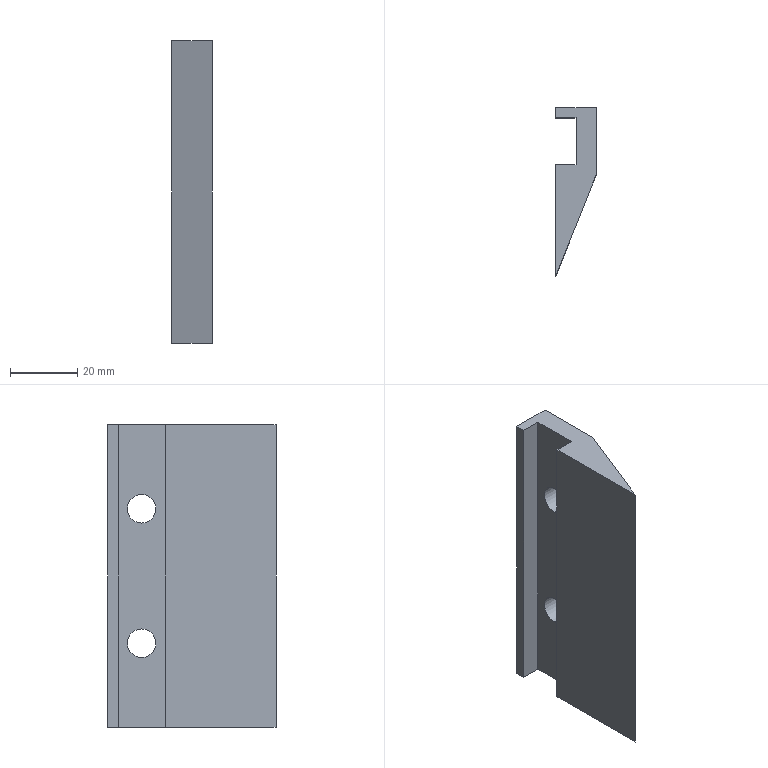Component | SolidWorks | HotKnife-Copy.1-1 | 1 solid | 14 faces | box 12 x 50 x 90 mm | volume 29559 mm3 | plane 10 | cylinder 4 | commonest cylinder face diameters 8.5 x4
build123d program:
from build123d import *

# Parameters (mm, degrees)
BOSS_EXTRUDE1_DEPTH            = 45
F_8_5_8_5_DIAMETER_HOLE1_D     = 8.5
F_8_5_8_5_DIAMETER_HOLE1_DEPTH = 80
F_8_5_8_5_DIAMETER_HOLE1_TIP   = 2.554
SKETCH4_W                      = 6
SKETCH4_H                      = 14
CUT_EXTRUDE1_DEPTH             = 66


with BuildPart() as part:
    # Sketch1 → Boss-Extrude1 (new, symmetric)
    with BuildSketch(Plane.XY):
        Polygon((0, -50), (0, 0), (12, 0), (12, -20), align=None)
    extrude(amount=BOSS_EXTRUDE1_DEPTH, both=True)

    # 8.5 _8.5_ Diameter Hole1
    with Locations(Plane(origin=(12, -32.177, 30.586), x_dir=(0, 0, 1), z_dir=(1, 0, 0))):
        with Locations((-50.586, -22.177), (-10.586, -22.177)):
            Hole(F_8_5_8_5_DIAMETER_HOLE1_D / 2, depth=F_8_5_8_5_DIAMETER_HOLE1_DEPTH)
            with Locations((0, 0, -(F_8_5_8_5_DIAMETER_HOLE1_DEPTH + F_8_5_8_5_DIAMETER_HOLE1_TIP / 2))):  # 118° drill point
                Cone(0, F_8_5_8_5_DIAMETER_HOLE1_D / 2, F_8_5_8_5_DIAMETER_HOLE1_TIP, mode=Mode.SUBTRACT)

    # Sketch4 → Cut-Extrude1 (cut, symmetric)
    with BuildSketch(Plane.XY):
        with Locations((3, -10)):
            Rectangle(SKETCH4_W, SKETCH4_H)
    extrude(amount=CUT_EXTRUDE1_DEPTH, both=True, mode=Mode.SUBTRACT)


solid = part.part

# Placed as in the assembly
solid = solid.moved(Location((-5.25, 201, 0), (0, 0, 0)))
STEP:
#1=COLOUR_RGB('',0.7922,0.8196,0.9333);
#2=FILL_AREA_STYLE_COLOUR('',#1);
#3=FILL_AREA_STYLE('',(#2));
#4=SURFACE_STYLE_FILL_AREA(#3);
#5=SURFACE_SIDE_STYLE('',(#4));
#6=SURFACE_STYLE_USAGE(.BOTH.,#5);
#7=PRESENTATION_STYLE_ASSIGNMENT((#6));
#8=CARTESIAN_POINT('',(0.02953,7.52,-0.9547));
#9=VERTEX_POINT('',#8);
#10=CARTESIAN_POINT('',(0.02953,7.52,-0.6201));
#11=VERTEX_POINT('',#10);
#12=CARTESIAN_POINT('',(0.02953,7.52,-0.7874));
#13=DIRECTION('',(-1.,-0.,0.));
#14=DIRECTION('',(-0.,1.,0.));
#15=AXIS2_PLACEMENT_3D('',#12,#13,#14);
#16=CIRCLE('',#15,0.1673);
#17=EDGE_CURVE('',#9,#11,#16,.T.);
#18=ORIENTED_EDGE('',*,*,#17,.T.);
#19=CARTESIAN_POINT('',(0.2657,7.52,-0.6201));
#20=VERTEX_POINT('',#19);
#21=CARTESIAN_POINT('',(0.2657,7.52,-0.6201));
#22=DIRECTION('',(1.,0.,0.));
#23=VECTOR('',#22,39.37);
#24=LINE('',#21,#23);
#25=EDGE_CURVE('',#11,#20,#24,.T.);
#26=ORIENTED_EDGE('',*,*,#25,.T.);
#27=CARTESIAN_POINT('',(0.2657,7.52,-0.9547));
#28=VERTEX_POINT('',#27);
#29=CARTESIAN_POINT('',(0.2657,7.52,-0.7874));
#30=DIRECTION('',(1.,0.,0.));
#31=DIRECTION('',(0.,0.,-1.));
#32=AXIS2_PLACEMENT_3D('',#29,#30,#31);
#33=CIRCLE('',#32,0.1673);
#34=EDGE_CURVE('',#20,#28,#33,.T.);
#35=ORIENTED_EDGE('',*,*,#34,.T.);
#36=CARTESIAN_POINT('',(0.2657,7.52,-0.9547));
#37=DIRECTION('',(1.,0.,0.));
#38=VECTOR('',#37,39.37);
#39=LINE('',#36,#38);
#40=EDGE_CURVE('',#9,#28,#39,.T.);
#41=ORIENTED_EDGE('',*,*,#40,.F.);
#42=EDGE_LOOP('',(#18,#26,#35,#41));
#43=FACE_OUTER_BOUND('',#42,.T.);
#44=CARTESIAN_POINT('',(0.2657,7.52,-0.7874));
#45=DIRECTION('',(1.,0.,0.));
#46=DIRECTION('',(0.,0.,-1.));
#47=AXIS2_PLACEMENT_3D('',#44,#45,#46);
#48=CYLINDRICAL_SURFACE('',#47,0.1673);
#49=ADVANCED_FACE('',(#43),#48,.F.);
#50=CARTESIAN_POINT('',(0.02953,7.52,0.6201));
#51=VERTEX_POINT('',#50);
#52=CARTESIAN_POINT('',(0.02953,7.52,0.9547));
#53=VERTEX_POINT('',#52);
#54=CARTESIAN_POINT('',(0.02953,7.52,0.7874));
#55=DIRECTION('',(-1.,-0.,0.));
#56=DIRECTION('',(-0.,1.,0.));
#57=AXIS2_PLACEMENT_3D('',#54,#55,#56);
#58=CIRCLE('',#57,0.1673);
#59=EDGE_CURVE('',#51,#53,#58,.T.);
#60=ORIENTED_EDGE('',*,*,#59,.T.);
#61=CARTESIAN_POINT('',(0.2657,7.52,0.9547));
#62=VERTEX_POINT('',#61);
#63=CARTESIAN_POINT('',(0.2657,7.52,0.9547));
#64=DIRECTION('',(1.,0.,0.));
#65=VECTOR('',#64,39.37);
#66=LINE('',#63,#65);
#67=EDGE_CURVE('',#53,#62,#66,.T.);
#68=ORIENTED_EDGE('',*,*,#67,.T.);
#69=CARTESIAN_POINT('',(0.2657,7.52,0.6201));
#70=VERTEX_POINT('',#69);
#71=CARTESIAN_POINT('',(0.2657,7.52,0.7874));
#72=DIRECTION('',(1.,0.,0.));
#73=DIRECTION('',(0.,0.,-1.));
#74=AXIS2_PLACEMENT_3D('',#71,#72,#73);
#75=CIRCLE('',#74,0.1673);
#76=EDGE_CURVE('',#62,#70,#75,.T.);
#77=ORIENTED_EDGE('',*,*,#76,.T.);
#78=CARTESIAN_POINT('',(0.2657,7.52,0.6201));
#79=DIRECTION('',(1.,0.,0.));
#80=VECTOR('',#79,39.37);
#81=LINE('',#78,#80);
#82=EDGE_CURVE('',#51,#70,#81,.T.);
#83=ORIENTED_EDGE('',*,*,#82,.F.);
#84=EDGE_LOOP('',(#60,#68,#77,#83));
#85=FACE_OUTER_BOUND('',#84,.T.);
#86=CARTESIAN_POINT('',(0.2657,7.52,0.7874));
#87=DIRECTION('',(1.,0.,0.));
#88=DIRECTION('',(0.,0.,-1.));
#89=AXIS2_PLACEMENT_3D('',#86,#87,#88);
#90=CYLINDRICAL_SURFACE('',#89,0.1673);
#91=ADVANCED_FACE('',(#85),#90,.F.);
#92=CARTESIAN_POINT('',(-0.2067,7.913,-1.772));
#93=VERTEX_POINT('',#92);
#94=CARTESIAN_POINT('',(-0.2067,7.795,-1.772));
#95=VERTEX_POINT('',#94);
#96=CARTESIAN_POINT('',(-0.2067,5.945,-1.772));
#97=DIRECTION('',(0.,-1.,0.));
#98=VECTOR('',#97,39.37);
#99=LINE('',#96,#98);
#100=EDGE_CURVE('',#93,#95,#99,.T.);
#101=ORIENTED_EDGE('',*,*,#100,.T.);
#102=CARTESIAN_POINT('',(-0.2067,7.795,1.772));
#103=VERTEX_POINT('',#102);
#104=CARTESIAN_POINT('',(-0.2067,7.795,-2.598));
#105=DIRECTION('',(0.,0.,1.));
#106=VECTOR('',#105,39.37);
#107=LINE('',#104,#106);
#108=EDGE_CURVE('',#95,#103,#107,.T.);
#109=ORIENTED_EDGE('',*,*,#108,.T.);
#110=CARTESIAN_POINT('',(-0.2067,7.913,1.772));
#111=VERTEX_POINT('',#110);
#112=CARTESIAN_POINT('',(-0.2067,5.945,1.772));
#113=DIRECTION('',(0.,-1.,0.));
#114=VECTOR('',#113,39.37);
#115=LINE('',#112,#114);
#116=EDGE_CURVE('',#111,#103,#115,.T.);
#117=ORIENTED_EDGE('',*,*,#116,.F.);
#118=CARTESIAN_POINT('',(-0.2067,7.913,1.772));
#119=DIRECTION('',(0.,0.,-1.));
#120=VECTOR('',#119,39.37);
#121=LINE('',#118,#120);
#122=EDGE_CURVE('',#111,#93,#121,.T.);
#123=ORIENTED_EDGE('',*,*,#122,.T.);
#124=EDGE_LOOP('',(#101,#109,#117,#123));
#125=FACE_OUTER_BOUND('',#124,.T.);
#126=CARTESIAN_POINT('',(-0.2067,5.945,1.772));
#127=DIRECTION('',(1.,0.,0.));
#128=DIRECTION('',(0.,0.,-1.));
#129=AXIS2_PLACEMENT_3D('',#126,#127,#128);
#130=PLANE('',#129);
#131=ADVANCED_FACE('',(#125),#130,.F.);
#132=CARTESIAN_POINT('',(0.2657,7.52,-0.7874));
#133=DIRECTION('',(1.,0.,0.));
#134=DIRECTION('',(0.,0.,-1.));
#135=AXIS2_PLACEMENT_3D('',#132,#133,#134);
#136=CIRCLE('',#135,0.1673);
#137=EDGE_CURVE('',#28,#20,#136,.T.);
#138=ORIENTED_EDGE('',*,*,#137,.F.);
#139=ORIENTED_EDGE('',*,*,#34,.F.);
#140=EDGE_LOOP('',(#138,#139));
#141=FACE_BOUND('',#140,.T.);
#142=CARTESIAN_POINT('',(0.2657,7.52,0.7874));
#143=DIRECTION('',(1.,0.,0.));
#144=DIRECTION('',(0.,0.,-1.));
#145=AXIS2_PLACEMENT_3D('',#142,#143,#144);
#146=CIRCLE('',#145,0.1673);
#147=EDGE_CURVE('',#70,#62,#146,.T.);
#148=ORIENTED_EDGE('',*,*,#147,.F.);
#149=ORIENTED_EDGE('',*,*,#76,.F.);
#150=EDGE_LOOP('',(#148,#149));
#151=FACE_BOUND('',#150,.T.);
#152=CARTESIAN_POINT('',(0.2657,7.126,-1.772));
#153=VERTEX_POINT('',#152);
#154=CARTESIAN_POINT('',(0.2657,7.913,-1.772));
#155=VERTEX_POINT('',#154);
#156=CARTESIAN_POINT('',(0.2657,7.913,-1.772));
#157=DIRECTION('',(-0.,1.,0.));
#158=VECTOR('',#157,39.37);
#159=LINE('',#156,#158);
#160=EDGE_CURVE('',#153,#155,#159,.T.);
#161=ORIENTED_EDGE('',*,*,#160,.T.);
#162=CARTESIAN_POINT('',(0.2657,7.913,1.772));
#163=VERTEX_POINT('',#162);
#164=CARTESIAN_POINT('',(0.2657,7.913,1.772));
#165=DIRECTION('',(0.,0.,-1.));
#166=VECTOR('',#165,39.37);
#167=LINE('',#164,#166);
#168=EDGE_CURVE('',#163,#155,#167,.T.);
#169=ORIENTED_EDGE('',*,*,#168,.F.);
#170=CARTESIAN_POINT('',(0.2657,7.126,1.772));
#171=VERTEX_POINT('',#170);
#172=CARTESIAN_POINT('',(0.2657,7.913,1.772));
#173=DIRECTION('',(-0.,1.,0.));
#174=VECTOR('',#173,39.37);
#175=LINE('',#172,#174);
#176=EDGE_CURVE('',#171,#163,#175,.T.);
#177=ORIENTED_EDGE('',*,*,#176,.F.);
#178=CARTESIAN_POINT('',(0.2657,7.126,1.772));
#179=DIRECTION('',(0.,0.,-1.));
#180=VECTOR('',#179,39.37);
#181=LINE('',#178,#180);
#182=EDGE_CURVE('',#171,#153,#181,.T.);
#183=ORIENTED_EDGE('',*,*,#182,.T.);
#184=EDGE_LOOP('',(#161,#169,#177,#183));
#185=FACE_OUTER_BOUND('',#184,.T.);
#186=CARTESIAN_POINT('',(0.2657,7.913,1.772));
#187=DIRECTION('',(-1.,-0.,0.));
#188=DIRECTION('',(0.,-1.,0.));
#189=AXIS2_PLACEMENT_3D('',#186,#187,#188);
#190=PLANE('',#189);
#191=ADVANCED_FACE('',(#141,#151,#185),#190,.F.);
#192=CARTESIAN_POINT('',(-0.2067,7.913,-1.772));
#193=DIRECTION('',(-1.,0.,0.));
#194=VECTOR('',#193,39.37);
#195=LINE('',#192,#194);
#196=EDGE_CURVE('',#155,#93,#195,.T.);
#197=ORIENTED_EDGE('',*,*,#196,.T.);
#198=ORIENTED_EDGE('',*,*,#122,.F.);
#199=CARTESIAN_POINT('',(-0.2067,7.913,1.772));
#200=DIRECTION('',(-1.,0.,0.));
#201=VECTOR('',#200,39.37);
#202=LINE('',#199,#201);
#203=EDGE_CURVE('',#163,#111,#202,.T.);
#204=ORIENTED_EDGE('',*,*,#203,.F.);
#205=ORIENTED_EDGE('',*,*,#168,.T.);
#206=EDGE_LOOP('',(#197,#198,#204,#205));
#207=FACE_OUTER_BOUND('',#206,.T.);
#208=CARTESIAN_POINT('',(-0.2067,7.913,1.772));
#209=DIRECTION('',(0.,-1.,0.));
#210=DIRECTION('',(0.,0.,-1.));
#211=AXIS2_PLACEMENT_3D('',#208,#209,#210);
#212=PLANE('',#211);
#213=ADVANCED_FACE('',(#207),#212,.F.);
#214=CARTESIAN_POINT('',(-0.2067,7.244,1.772));
#215=VERTEX_POINT('',#214);
#216=CARTESIAN_POINT('',(-0.2067,5.945,1.772));
#217=VERTEX_POINT('',#216);
#218=CARTESIAN_POINT('',(-0.2067,5.945,1.772));
#219=DIRECTION('',(0.,-1.,0.));
#220=VECTOR('',#219,39.37);
#221=LINE('',#218,#220);
#222=EDGE_CURVE('',#215,#217,#221,.T.);
#223=ORIENTED_EDGE('',*,*,#222,.F.);
#224=CARTESIAN_POINT('',(-0.2067,7.244,-1.772));
#225=VERTEX_POINT('',#224);
#226=CARTESIAN_POINT('',(-0.2067,7.244,-2.598));
#227=DIRECTION('',(0.,0.,1.));
#228=VECTOR('',#227,39.37);
#229=LINE('',#226,#228);
#230=EDGE_CURVE('',#225,#215,#229,.T.);
#231=ORIENTED_EDGE('',*,*,#230,.F.);
#232=CARTESIAN_POINT('',(-0.2067,5.945,-1.772));
#233=VERTEX_POINT('',#232);
#234=CARTESIAN_POINT('',(-0.2067,5.945,-1.772));
#235=DIRECTION('',(0.,-1.,0.));
#236=VECTOR('',#235,39.37);
#237=LINE('',#234,#236);
#238=EDGE_CURVE('',#225,#233,#237,.T.);
#239=ORIENTED_EDGE('',*,*,#238,.T.);
#240=CARTESIAN_POINT('',(-0.2067,5.945,1.772));
#241=DIRECTION('',(0.,0.,-1.));
#242=VECTOR('',#241,39.37);
#243=LINE('',#240,#242);
#244=EDGE_CURVE('',#217,#233,#243,.T.);
#245=ORIENTED_EDGE('',*,*,#244,.F.);
#246=EDGE_LOOP('',(#223,#231,#239,#245));
#247=FACE_OUTER_BOUND('',#246,.T.);
#248=CARTESIAN_POINT('',(-0.2067,5.945,1.772));
#249=DIRECTION('',(1.,0.,0.));
#250=DIRECTION('',(0.,0.,-1.));
#251=AXIS2_PLACEMENT_3D('',#248,#249,#250);
#252=PLANE('',#251);
#253=ADVANCED_FACE('',(#247),#252,.F.);
#254=CARTESIAN_POINT('',(0.2657,7.126,-1.772));
#255=DIRECTION('',(0.3714,0.9285,0.));
#256=VECTOR('',#255,39.37);
#257=LINE('',#254,#256);
#258=EDGE_CURVE('',#233,#153,#257,.T.);
#259=ORIENTED_EDGE('',*,*,#258,.T.);
#260=ORIENTED_EDGE('',*,*,#182,.F.);
#261=CARTESIAN_POINT('',(0.2657,7.126,1.772));
#262=DIRECTION('',(0.3714,0.9285,0.));
#263=VECTOR('',#262,39.37);
#264=LINE('',#261,#263);
#265=EDGE_CURVE('',#217,#171,#264,.T.);
#266=ORIENTED_EDGE('',*,*,#265,.F.);
#267=ORIENTED_EDGE('',*,*,#244,.T.);
#268=EDGE_LOOP('',(#259,#260,#266,#267));
#269=FACE_OUTER_BOUND('',#268,.T.);
#270=CARTESIAN_POINT('',(0.2657,7.126,1.772));
#271=DIRECTION('',(-0.9285,0.3714,0.));
#272=DIRECTION('',(-0.3714,-0.9285,0.));
#273=AXIS2_PLACEMENT_3D('',#270,#271,#272);
#274=PLANE('',#273);
#275=ADVANCED_FACE('',(#269),#274,.F.);
#276=CARTESIAN_POINT('',(0.02953,7.795,1.772));
#277=VERTEX_POINT('',#276);
#278=CARTESIAN_POINT('',(0.2657,7.795,1.772));
#279=DIRECTION('',(-1.,0.,0.));
#280=VECTOR('',#279,39.37);
#281=LINE('',#278,#280);
#282=EDGE_CURVE('',#277,#103,#281,.T.);
#283=ORIENTED_EDGE('',*,*,#282,.F.);
#284=CARTESIAN_POINT('',(0.02953,7.244,1.772));
#285=VERTEX_POINT('',#284);
#286=CARTESIAN_POINT('',(0.02953,7.913,1.772));
#287=DIRECTION('',(-0.,1.,0.));
#288=VECTOR('',#287,39.37);
#289=LINE('',#286,#288);
#290=EDGE_CURVE('',#285,#277,#289,.T.);
#291=ORIENTED_EDGE('',*,*,#290,.F.);
#292=CARTESIAN_POINT('',(0.2657,7.244,1.772));
#293=DIRECTION('',(1.,0.,0.));
#294=VECTOR('',#293,39.37);
#295=LINE('',#292,#294);
#296=EDGE_CURVE('',#215,#285,#295,.T.);
#297=ORIENTED_EDGE('',*,*,#296,.F.);
#298=ORIENTED_EDGE('',*,*,#222,.T.);
#299=ORIENTED_EDGE('',*,*,#265,.T.);
#300=ORIENTED_EDGE('',*,*,#176,.T.);
#301=ORIENTED_EDGE('',*,*,#203,.T.);
#302=ORIENTED_EDGE('',*,*,#116,.T.);
#303=EDGE_LOOP('',(#283,#291,#297,#298,#299,#300,#301,#302));
#304=FACE_OUTER_BOUND('',#303,.T.);
#305=CARTESIAN_POINT('',(0.2657,7.913,1.772));
#306=DIRECTION('',(0.,0.,1.));
#307=DIRECTION('',(1.,0.,0.));
#308=AXIS2_PLACEMENT_3D('',#305,#306,#307);
#309=PLANE('',#308);
#310=ADVANCED_FACE('',(#304),#309,.T.);
#311=CARTESIAN_POINT('',(0.02953,7.244,-1.772));
#312=VERTEX_POINT('',#311);
#313=CARTESIAN_POINT('',(0.02953,7.795,-1.772));
#314=VERTEX_POINT('',#313);
#315=CARTESIAN_POINT('',(0.02953,7.913,-1.772));
#316=DIRECTION('',(-0.,1.,0.));
#317=VECTOR('',#316,39.37);
#318=LINE('',#315,#317);
#319=EDGE_CURVE('',#312,#314,#318,.T.);
#320=ORIENTED_EDGE('',*,*,#319,.T.);
#321=CARTESIAN_POINT('',(0.2657,7.795,-1.772));
#322=DIRECTION('',(-1.,0.,0.));
#323=VECTOR('',#322,39.37);
#324=LINE('',#321,#323);
#325=EDGE_CURVE('',#314,#95,#324,.T.);
#326=ORIENTED_EDGE('',*,*,#325,.T.);
#327=ORIENTED_EDGE('',*,*,#100,.F.);
#328=ORIENTED_EDGE('',*,*,#196,.F.);
#329=ORIENTED_EDGE('',*,*,#160,.F.);
#330=ORIENTED_EDGE('',*,*,#258,.F.);
#331=ORIENTED_EDGE('',*,*,#238,.F.);
#332=CARTESIAN_POINT('',(0.2657,7.244,-1.772));
#333=DIRECTION('',(1.,0.,0.));
#334=VECTOR('',#333,39.37);
#335=LINE('',#332,#334);
#336=EDGE_CURVE('',#225,#312,#335,.T.);
#337=ORIENTED_EDGE('',*,*,#336,.T.);
#338=EDGE_LOOP('',(#320,#326,#327,#328,#329,#330,#331,#337));
#339=FACE_OUTER_BOUND('',#338,.T.);
#340=CARTESIAN_POINT('',(0.2657,7.913,-1.772));
#341=DIRECTION('',(0.,0.,1.));
#342=DIRECTION('',(1.,0.,0.));
#343=AXIS2_PLACEMENT_3D('',#340,#341,#342);
#344=PLANE('',#343);
#345=ADVANCED_FACE('',(#339),#344,.F.);
#346=ORIENTED_EDGE('',*,*,#67,.F.);
#347=CARTESIAN_POINT('',(0.02953,7.52,0.7874));
#348=DIRECTION('',(-1.,-0.,0.));
#349=DIRECTION('',(-0.,1.,0.));
#350=AXIS2_PLACEMENT_3D('',#347,#348,#349);
#351=CIRCLE('',#350,0.1673);
#352=EDGE_CURVE('',#53,#51,#351,.T.);
#353=ORIENTED_EDGE('',*,*,#352,.T.);
#354=ORIENTED_EDGE('',*,*,#82,.T.);
#355=ORIENTED_EDGE('',*,*,#147,.T.);
#356=EDGE_LOOP('',(#346,#353,#354,#355));
#357=FACE_OUTER_BOUND('',#356,.T.);
#358=CARTESIAN_POINT('',(0.2657,7.52,0.7874));
#359=DIRECTION('',(1.,0.,0.));
#360=DIRECTION('',(0.,0.,-1.));
#361=AXIS2_PLACEMENT_3D('',#358,#359,#360);
#362=CYLINDRICAL_SURFACE('',#361,0.1673);
#363=ADVANCED_FACE('',(#357),#362,.F.);
#364=ORIENTED_EDGE('',*,*,#25,.F.);
#365=CARTESIAN_POINT('',(0.02953,7.52,-0.7874));
#366=DIRECTION('',(-1.,-0.,0.));
#367=DIRECTION('',(-0.,1.,0.));
#368=AXIS2_PLACEMENT_3D('',#365,#366,#367);
#369=CIRCLE('',#368,0.1673);
#370=EDGE_CURVE('',#11,#9,#369,.T.);
#371=ORIENTED_EDGE('',*,*,#370,.T.);
#372=ORIENTED_EDGE('',*,*,#40,.T.);
#373=ORIENTED_EDGE('',*,*,#137,.T.);
#374=EDGE_LOOP('',(#364,#371,#372,#373));
#375=FACE_OUTER_BOUND('',#374,.T.);
#376=CARTESIAN_POINT('',(0.2657,7.52,-0.7874));
#377=DIRECTION('',(1.,0.,0.));
#378=DIRECTION('',(0.,0.,-1.));
#379=AXIS2_PLACEMENT_3D('',#376,#377,#378);
#380=CYLINDRICAL_SURFACE('',#379,0.1673);
#381=ADVANCED_FACE('',(#375),#380,.F.);
#382=ORIENTED_EDGE('',*,*,#282,.T.);
#383=ORIENTED_EDGE('',*,*,#108,.F.);
#384=ORIENTED_EDGE('',*,*,#325,.F.);
#385=CARTESIAN_POINT('',(0.02953,7.795,-2.598));
#386=DIRECTION('',(0.,0.,1.));
#387=VECTOR('',#386,39.37);
#388=LINE('',#385,#387);
#389=EDGE_CURVE('',#314,#277,#388,.T.);
#390=ORIENTED_EDGE('',*,*,#389,.T.);
#391=EDGE_LOOP('',(#382,#383,#384,#390));
#392=FACE_OUTER_BOUND('',#391,.T.);
#393=CARTESIAN_POINT('',(-0.2067,7.795,-2.598));
#394=DIRECTION('',(0.,1.,0.));
#395=DIRECTION('',(0.,0.,1.));
#396=AXIS2_PLACEMENT_3D('',#393,#394,#395);
#397=PLANE('',#396);
#398=ADVANCED_FACE('',(#392),#397,.F.);
#399=ORIENTED_EDGE('',*,*,#296,.T.);
#400=CARTESIAN_POINT('',(0.02953,7.244,-2.598));
#401=DIRECTION('',(0.,0.,1.));
#402=VECTOR('',#401,39.37);
#403=LINE('',#400,#402);
#404=EDGE_CURVE('',#312,#285,#403,.T.);
#405=ORIENTED_EDGE('',*,*,#404,.F.);
#406=ORIENTED_EDGE('',*,*,#336,.F.);
#407=ORIENTED_EDGE('',*,*,#230,.T.);
#408=EDGE_LOOP('',(#399,#405,#406,#407));
#409=FACE_OUTER_BOUND('',#408,.T.);
#410=CARTESIAN_POINT('',(-0.2067,7.244,-2.598));
#411=DIRECTION('',(0.,-1.,0.));
#412=DIRECTION('',(0.,0.,-1.));
#413=AXIS2_PLACEMENT_3D('',#410,#411,#412);
#414=PLANE('',#413);
#415=ADVANCED_FACE('',(#409),#414,.F.);
#416=ORIENTED_EDGE('',*,*,#290,.T.);
#417=ORIENTED_EDGE('',*,*,#389,.F.);
#418=ORIENTED_EDGE('',*,*,#319,.F.);
#419=ORIENTED_EDGE('',*,*,#404,.T.);
#420=EDGE_LOOP('',(#416,#417,#418,#419));
#421=FACE_OUTER_BOUND('',#420,.T.);
#422=ORIENTED_EDGE('',*,*,#59,.F.);
#423=ORIENTED_EDGE('',*,*,#352,.F.);
#424=EDGE_LOOP('',(#422,#423));
#425=FACE_BOUND('',#424,.T.);
#426=ORIENTED_EDGE('',*,*,#17,.F.);
#427=ORIENTED_EDGE('',*,*,#370,.F.);
#428=EDGE_LOOP('',(#426,#427));
#429=FACE_BOUND('',#428,.T.);
#430=CARTESIAN_POINT('',(0.02953,7.795,-2.598));
#431=DIRECTION('',(1.,0.,0.));
#432=DIRECTION('',(-0.,1.,0.));
#433=AXIS2_PLACEMENT_3D('',#430,#431,#432);
#434=PLANE('',#433);
#435=ADVANCED_FACE('',(#421,#425,#429),#434,.F.);
#436=CLOSED_SHELL('',(#49,#91,#131,#191,#213,#253,#275,#310,#345,#363,#381,#398,#415,#435));
#437=MANIFOLD_SOLID_BREP('',#436);
#438=STYLED_ITEM('',(#7),#437);
#439=PRESENTATION_LAYER_ASSIGNMENT('','',(#438));
#440=CARTESIAN_POINT('',(0.,0.,0.));
#441=DIRECTION('',(0.,0.,1.));
#442=DIRECTION('',(1.,0.,0.));
#443=AXIS2_PLACEMENT_3D('',#440,#441,#442);
#444=(LENGTH_UNIT()NAMED_UNIT(*)SI_UNIT($,.METRE.));
#445=LENGTH_MEASURE_WITH_UNIT(LENGTH_MEASURE(0.0254),#444);
#446=DIMENSIONAL_EXPONENTS(1.,0.,0.,0.,0.,0.,0.);
#447=(CONVERSION_BASED_UNIT('',#445)LENGTH_UNIT()NAMED_UNIT(#446));
#448=UNCERTAINTY_MEASURE_WITH_UNIT(LENGTH_MEASURE(0.00001),#447,'','');
#449=(NAMED_UNIT(*)PLANE_ANGLE_UNIT()SI_UNIT($,.RADIAN.));
#450=(NAMED_UNIT(*)SI_UNIT($,.STERADIAN.)SOLID_ANGLE_UNIT());
#451=(GEOMETRIC_REPRESENTATION_CONTEXT(3)GLOBAL_UNCERTAINTY_ASSIGNED_CONTEXT((#448))GLOBAL_UNIT_ASSIGNED_CONTEXT((#447,#449,#450))REPRESENTATION_CONTEXT('',''));
#452=ADVANCED_BREP_SHAPE_REPRESENTATION('',(#437,#443),#451);
#453=(LENGTH_UNIT()NAMED_UNIT(*)SI_UNIT($,.METRE.));
#454=LENGTH_MEASURE_WITH_UNIT(LENGTH_MEASURE(0.0254),#453);
#455=DIMENSIONAL_EXPONENTS(1.,0.,0.,0.,0.,0.,0.);
#456=(CONVERSION_BASED_UNIT('',#454)LENGTH_UNIT()NAMED_UNIT(#455));
#457=UNCERTAINTY_MEASURE_WITH_UNIT(LENGTH_MEASURE(0.00001),#456,'','');
#458=(NAMED_UNIT(*)PLANE_ANGLE_UNIT()SI_UNIT($,.RADIAN.));
#459=(NAMED_UNIT(*)SI_UNIT($,.STERADIAN.)SOLID_ANGLE_UNIT());
#460=(GEOMETRIC_REPRESENTATION_CONTEXT(3)GLOBAL_UNCERTAINTY_ASSIGNED_CONTEXT((#457))GLOBAL_UNIT_ASSIGNED_CONTEXT((#456,#458,#459))REPRESENTATION_CONTEXT('',''));
#461=MECHANICAL_DESIGN_GEOMETRIC_PRESENTATION_REPRESENTATION('',(#438),#460);